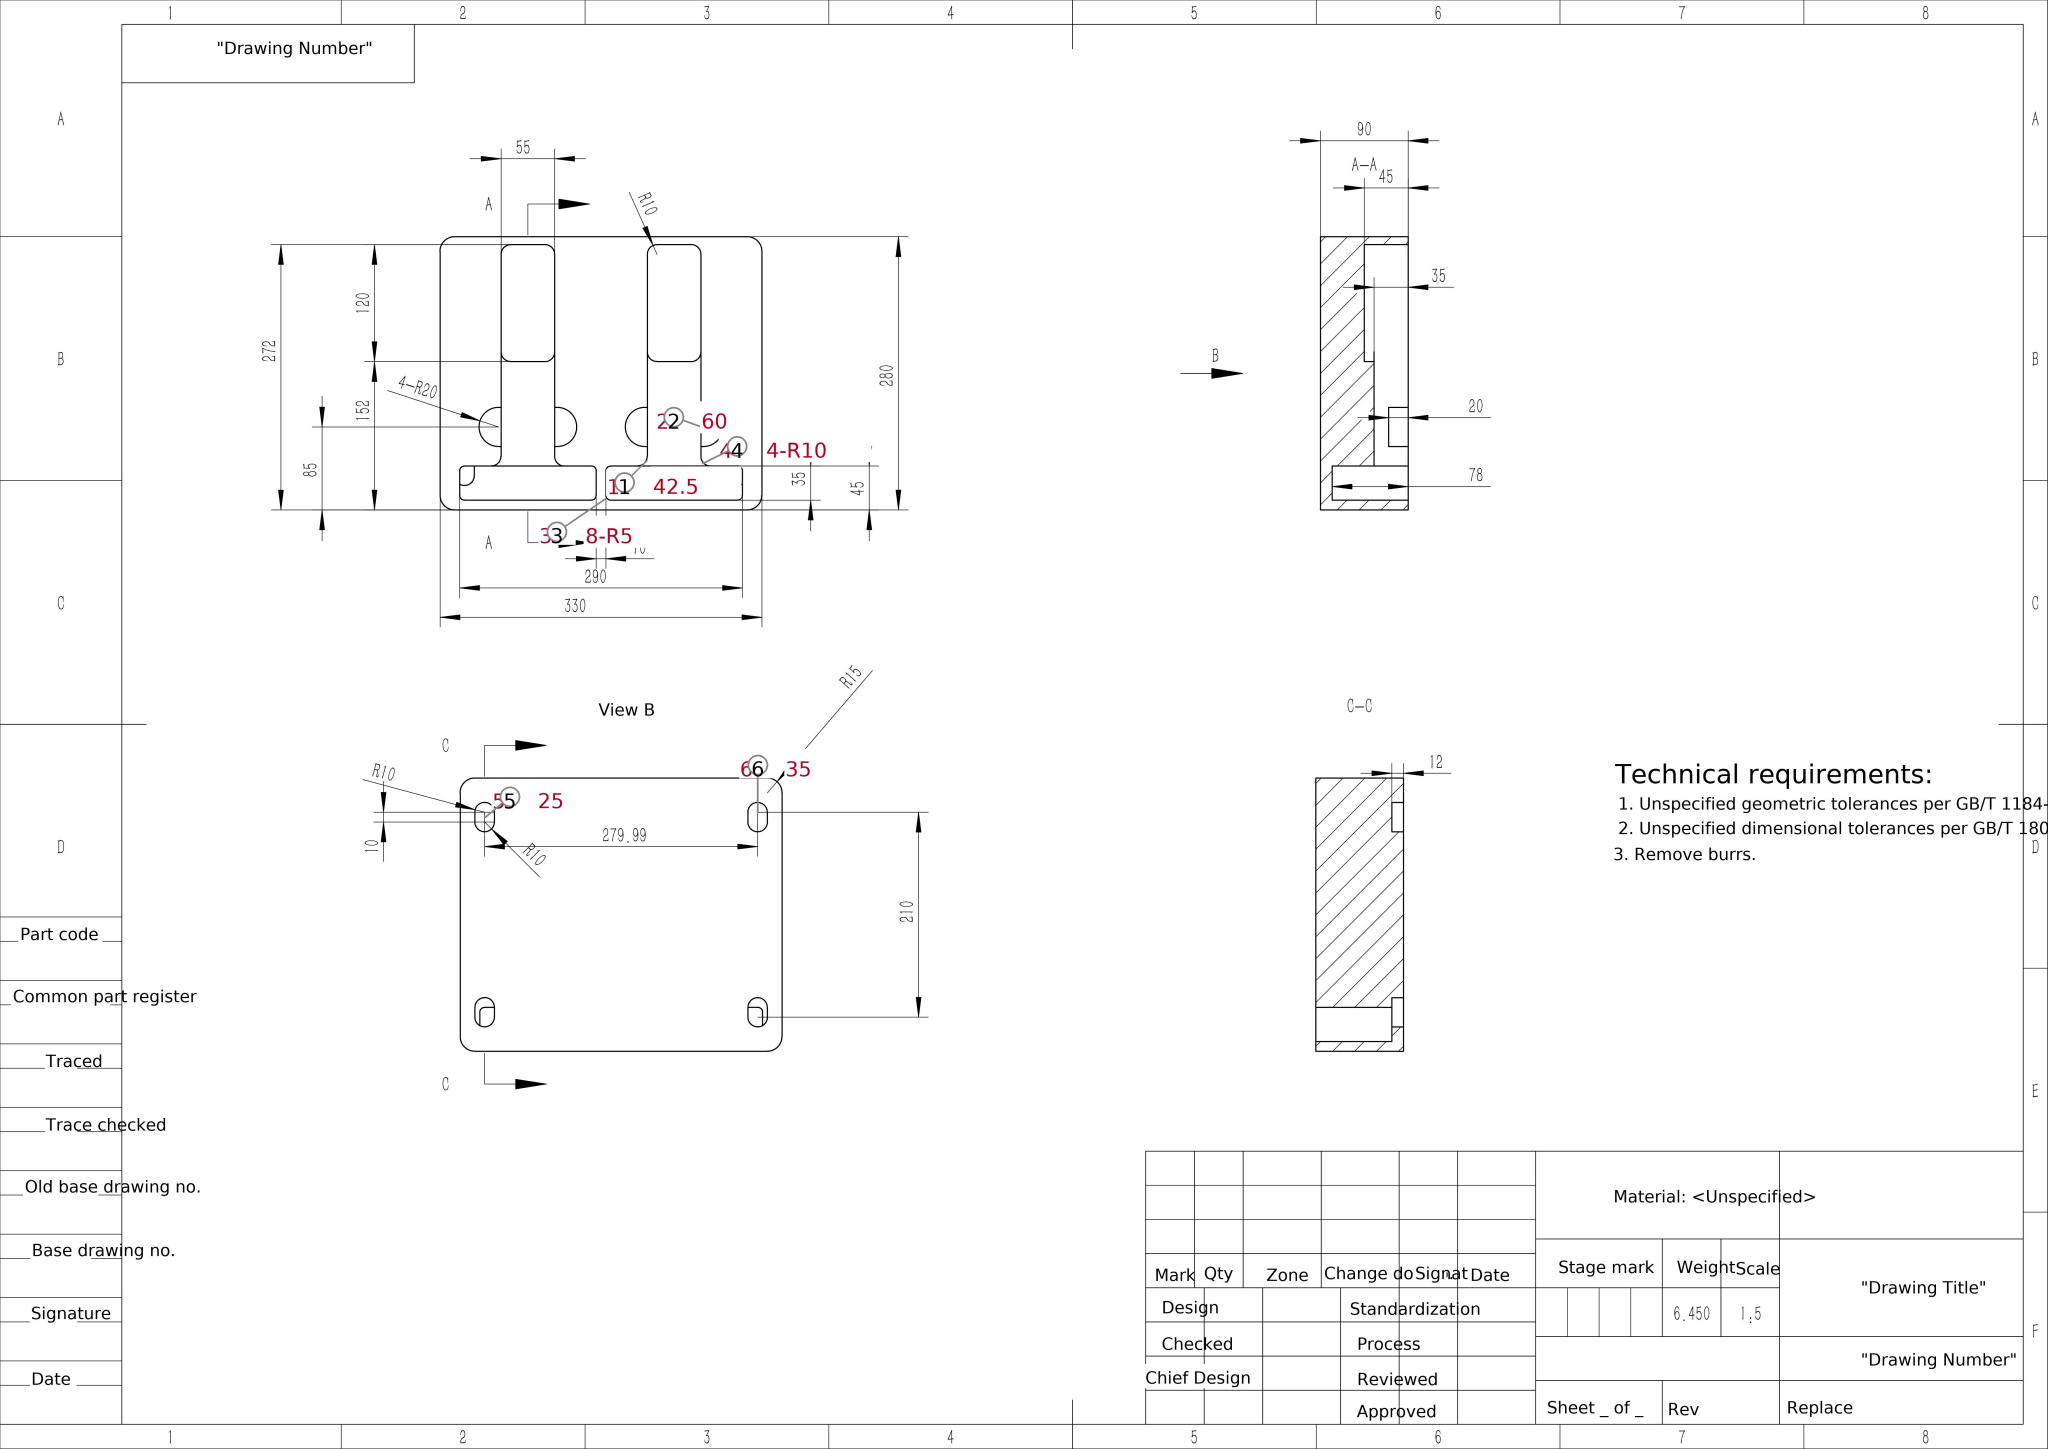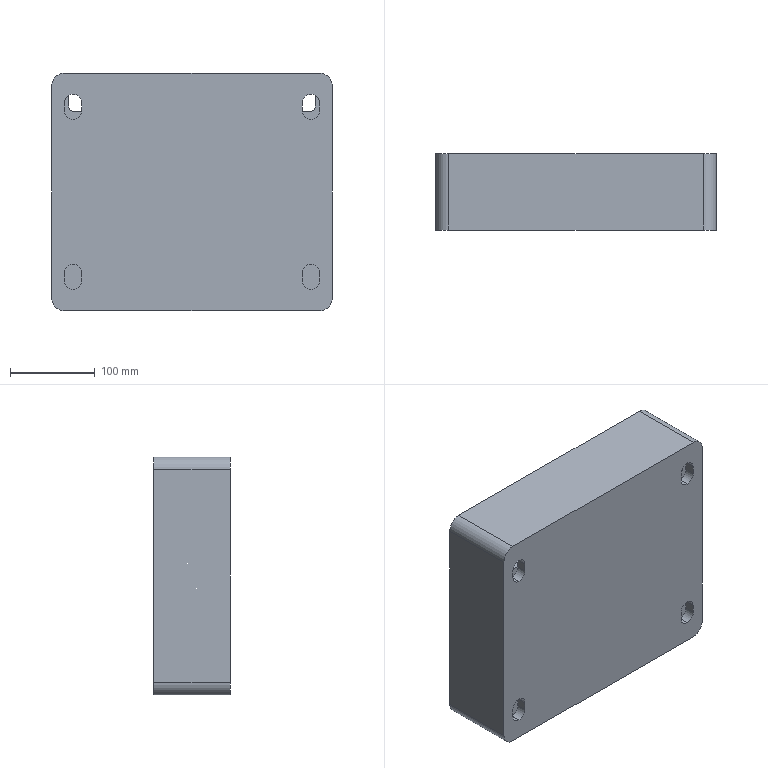Part | SolidWorks | mm | 1 solid | 92 faces | box 330 x 90 x 280 mm | volume 6450387 mm3 | plane 52 | cylinder 40 | commonest cylinder face diameters 20 x24 10 x8 40 x4 30 x4